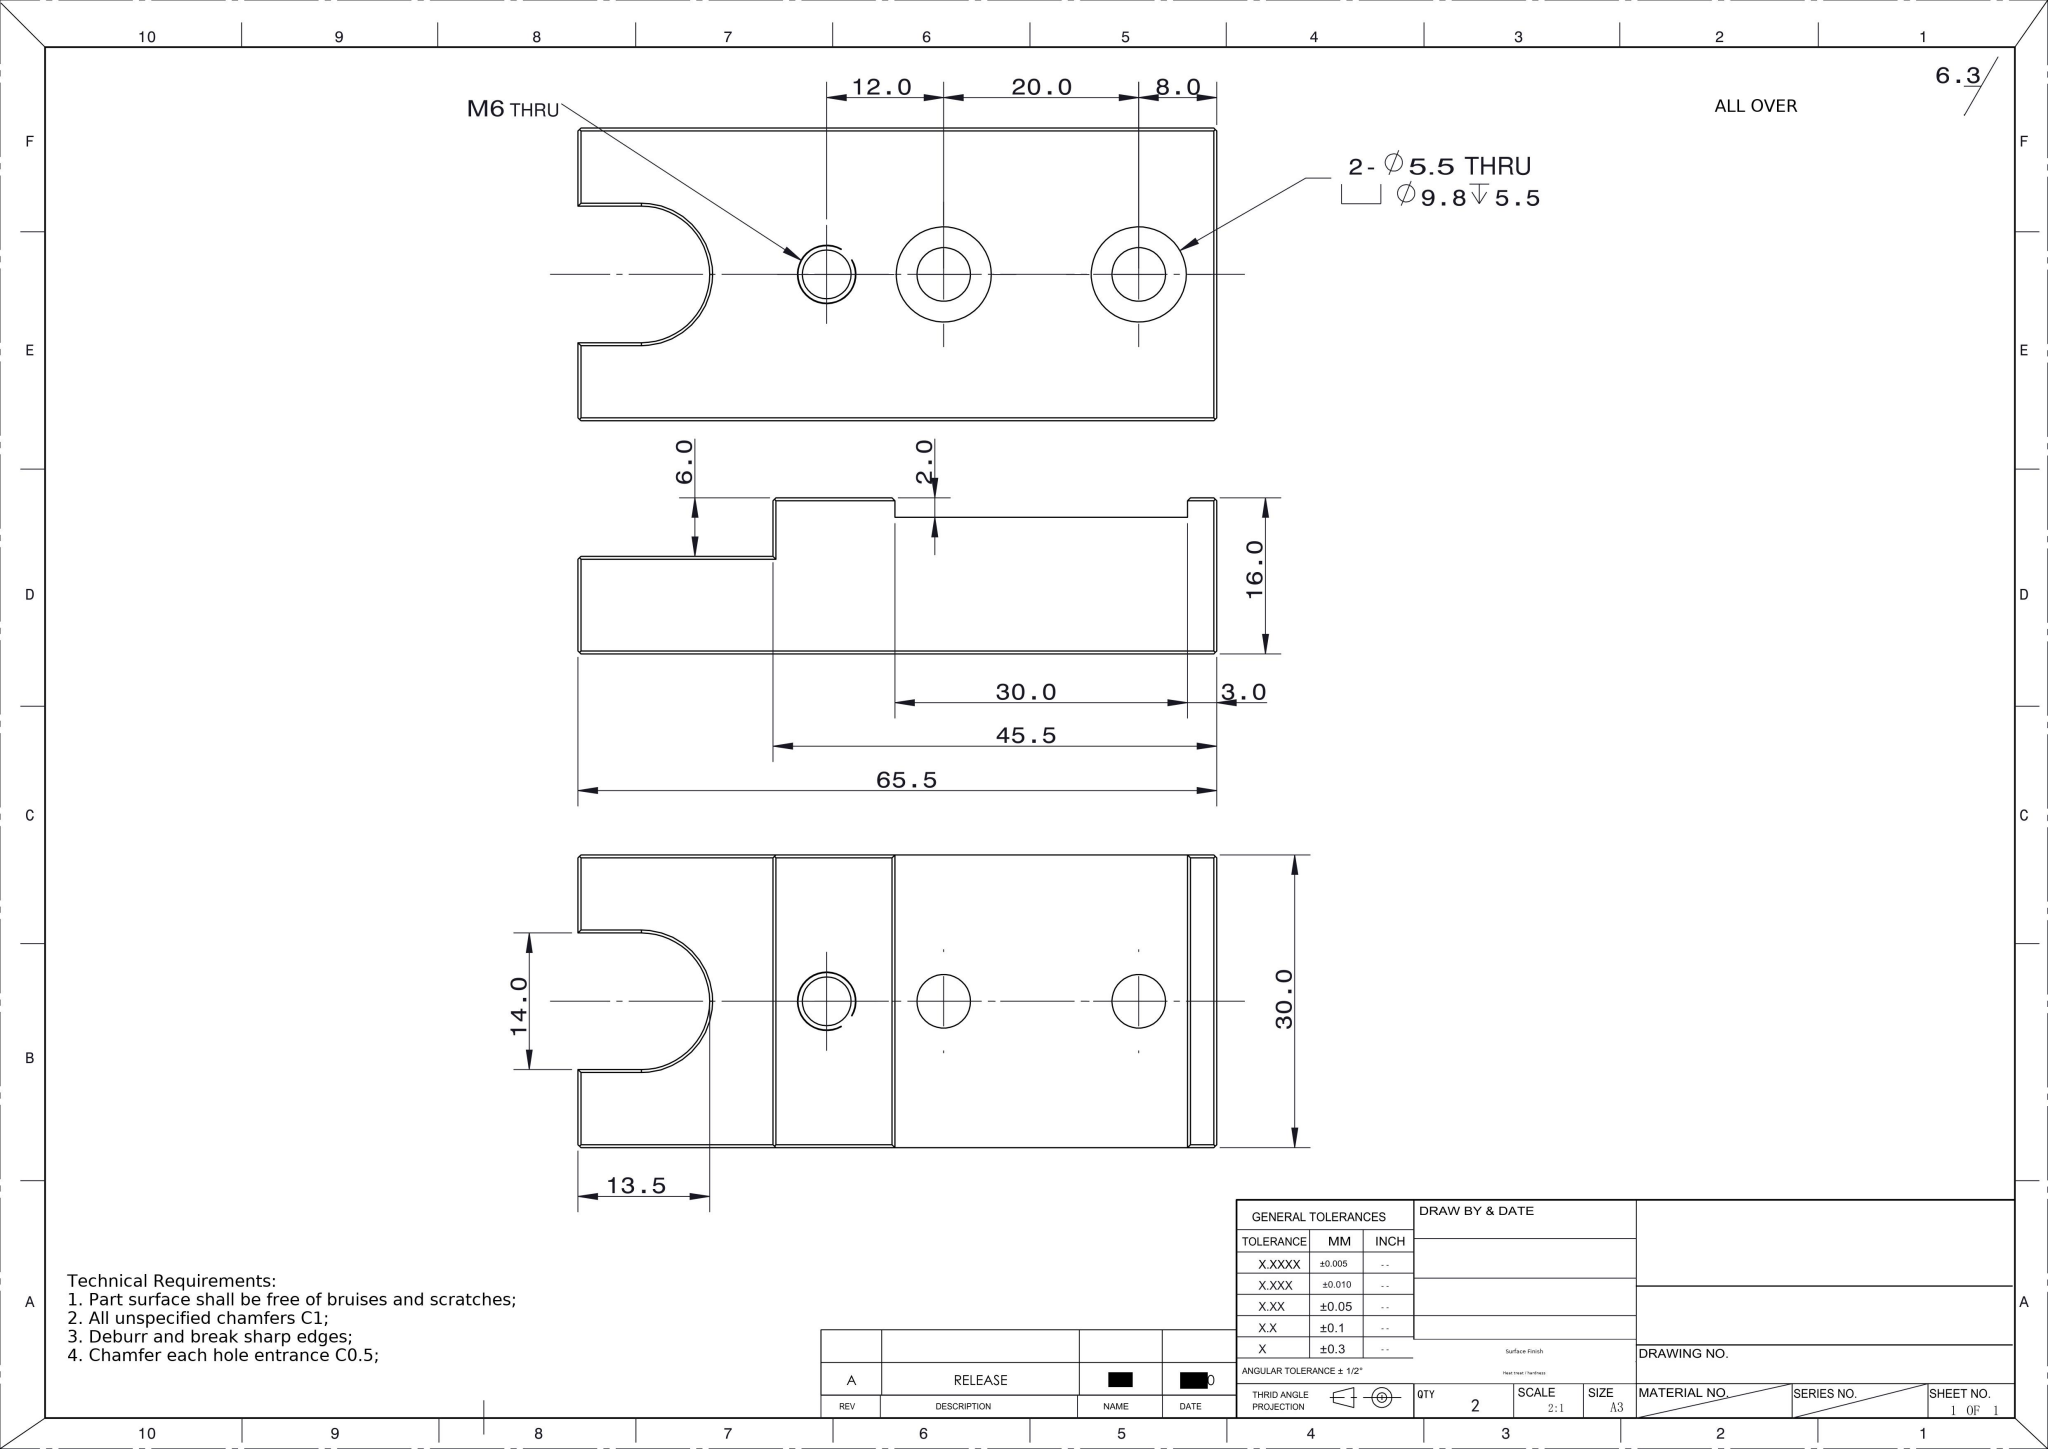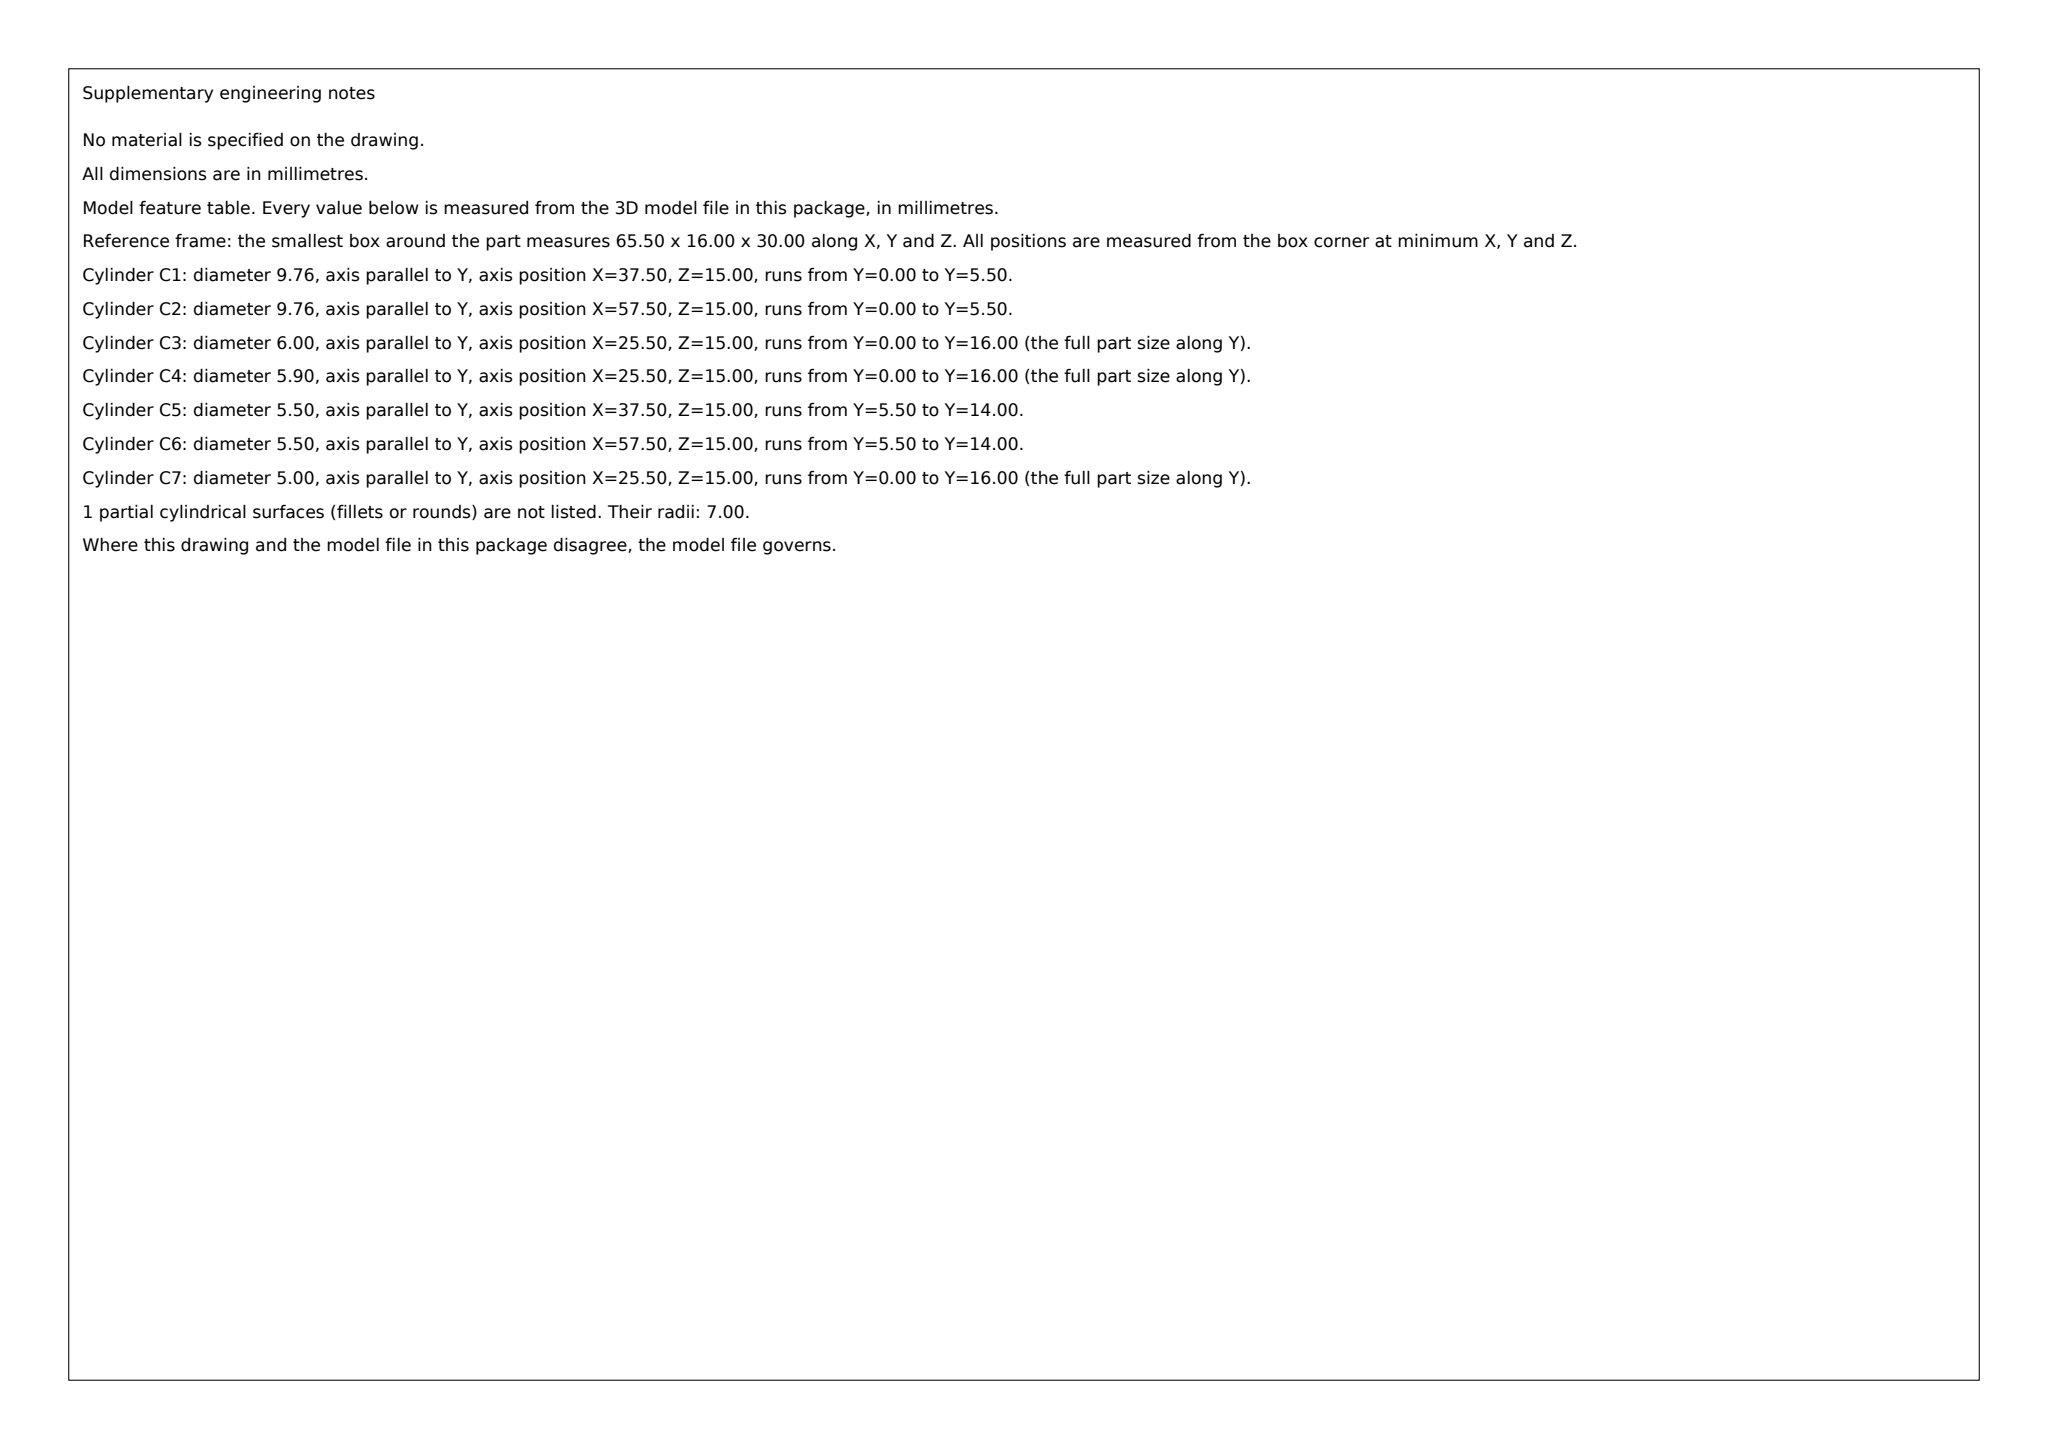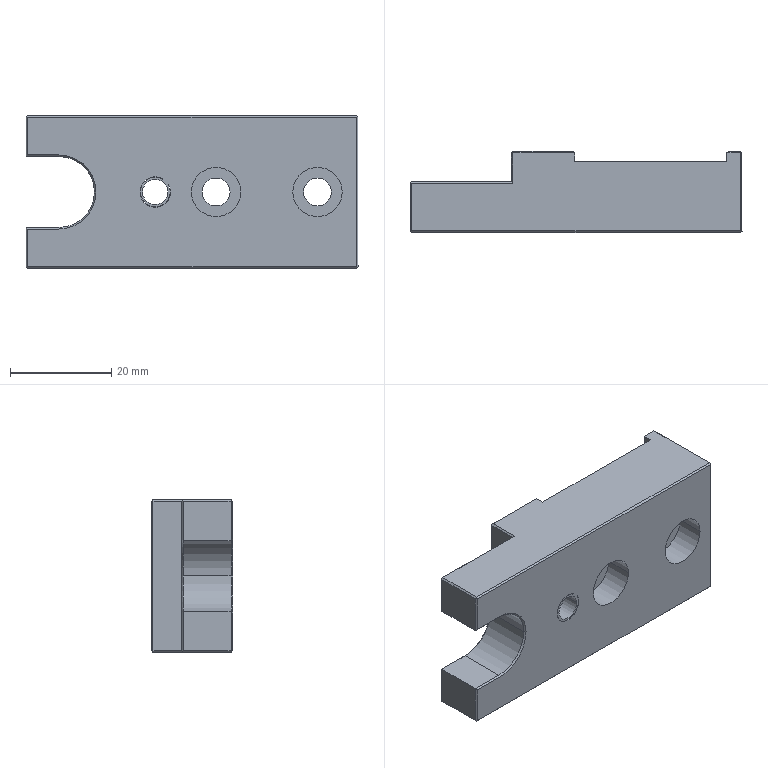Part | SolidWorks | mm | 1 solid | 68 faces | box 65.5 x 16 x 30 mm | volume 22784 mm3 | plane 46 | cylinder 18 | spline 4 | commonest cylinder face diameters 9.75 x4 5.5 x4 5.9 x3 6 x3 5 x2 14 x2